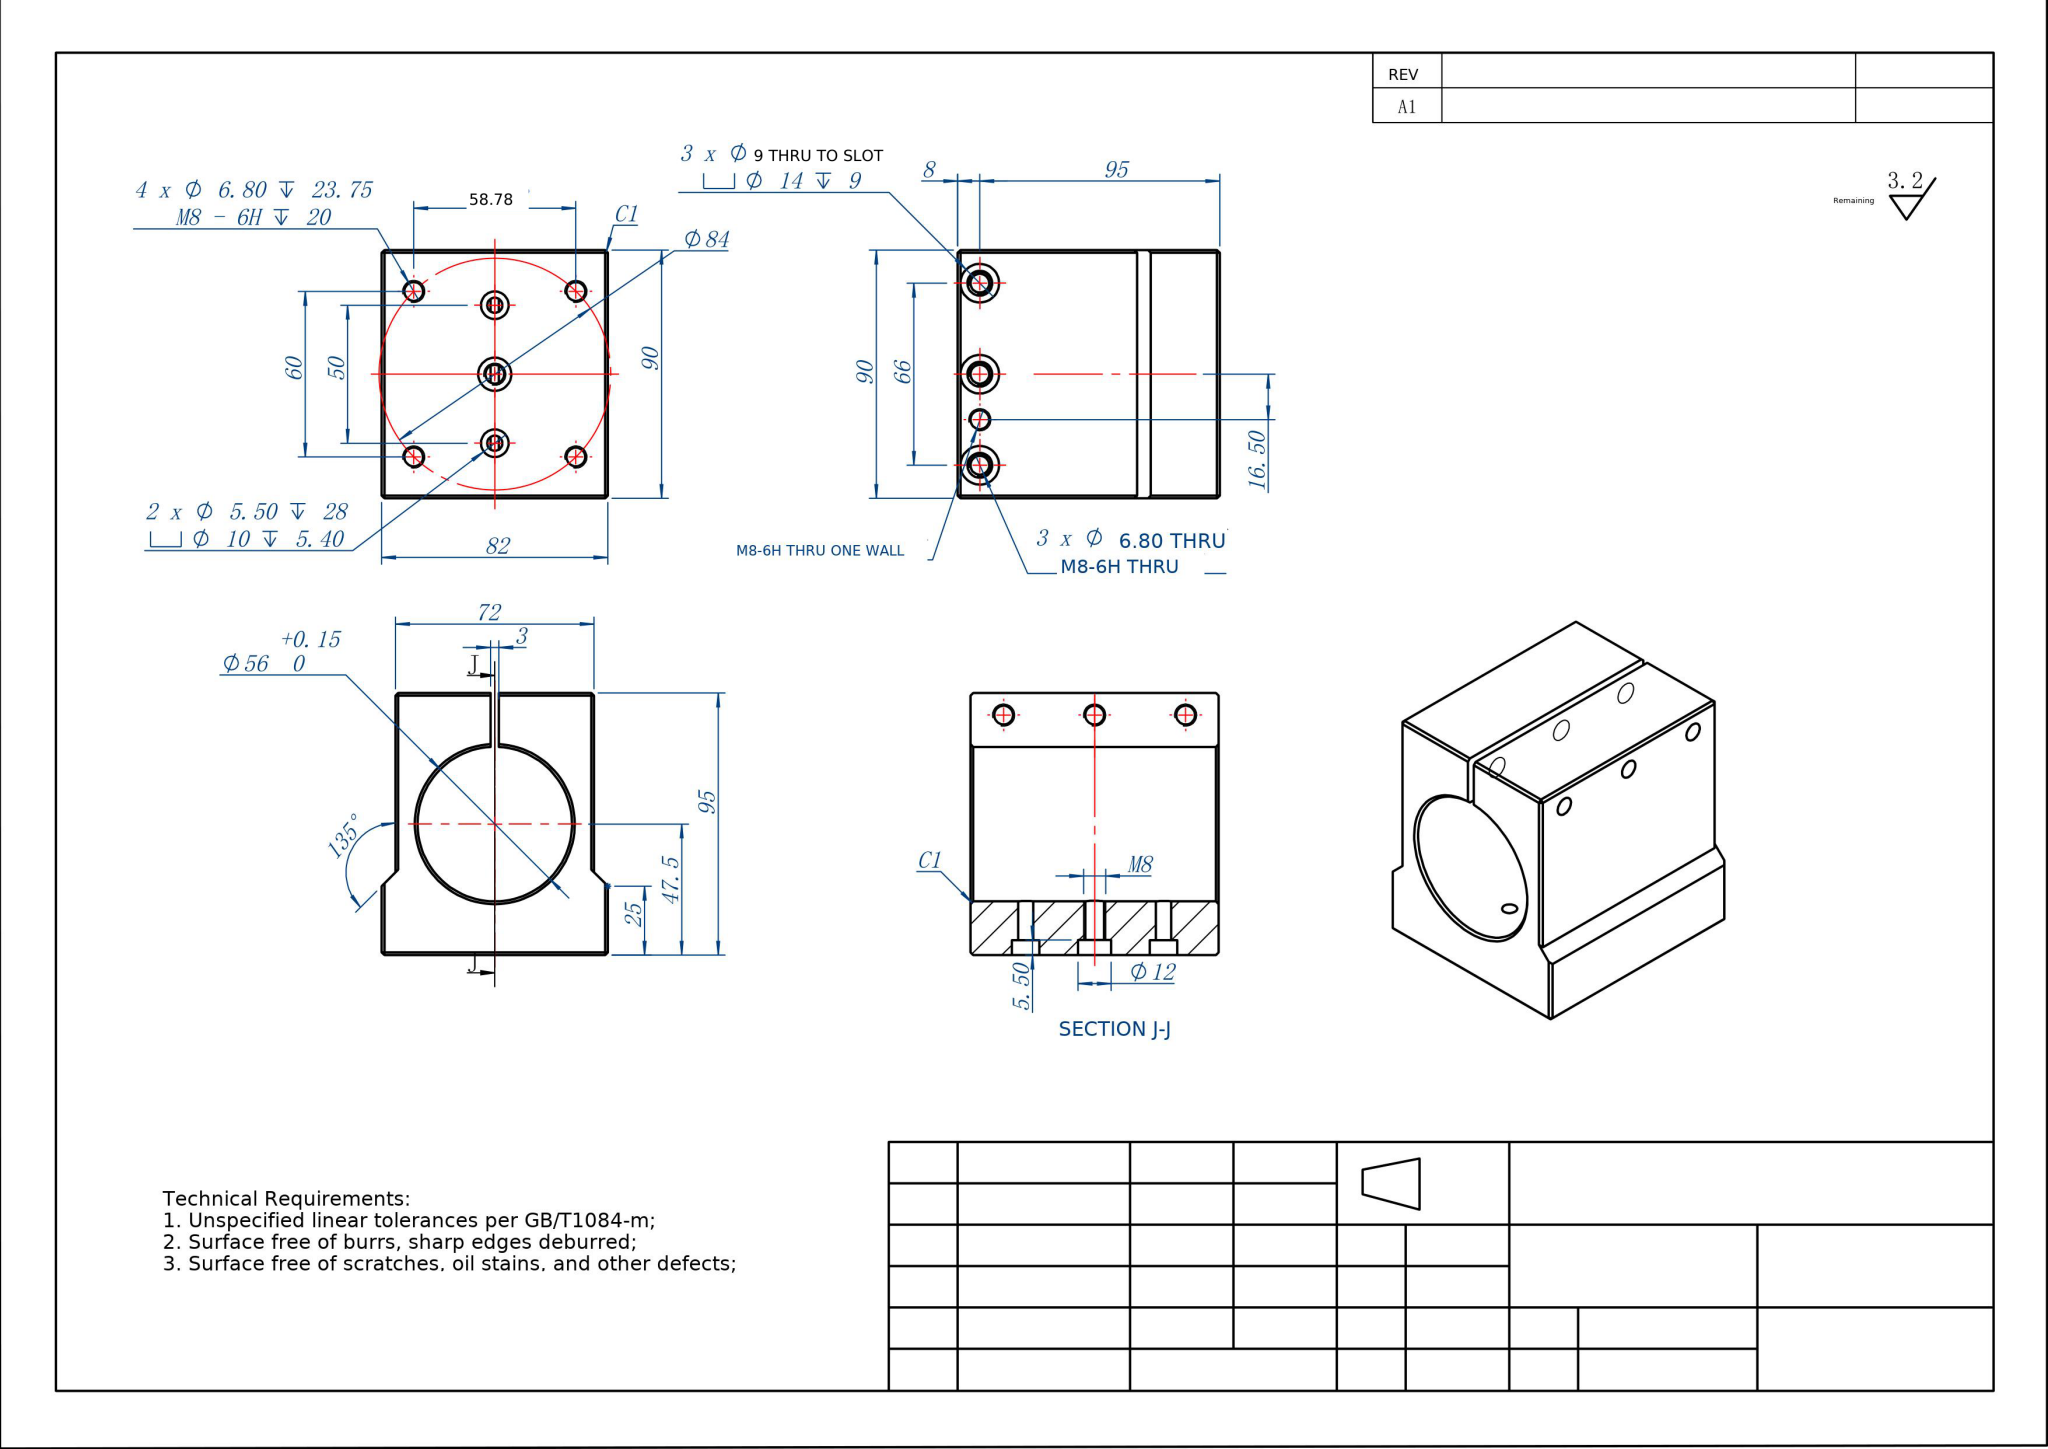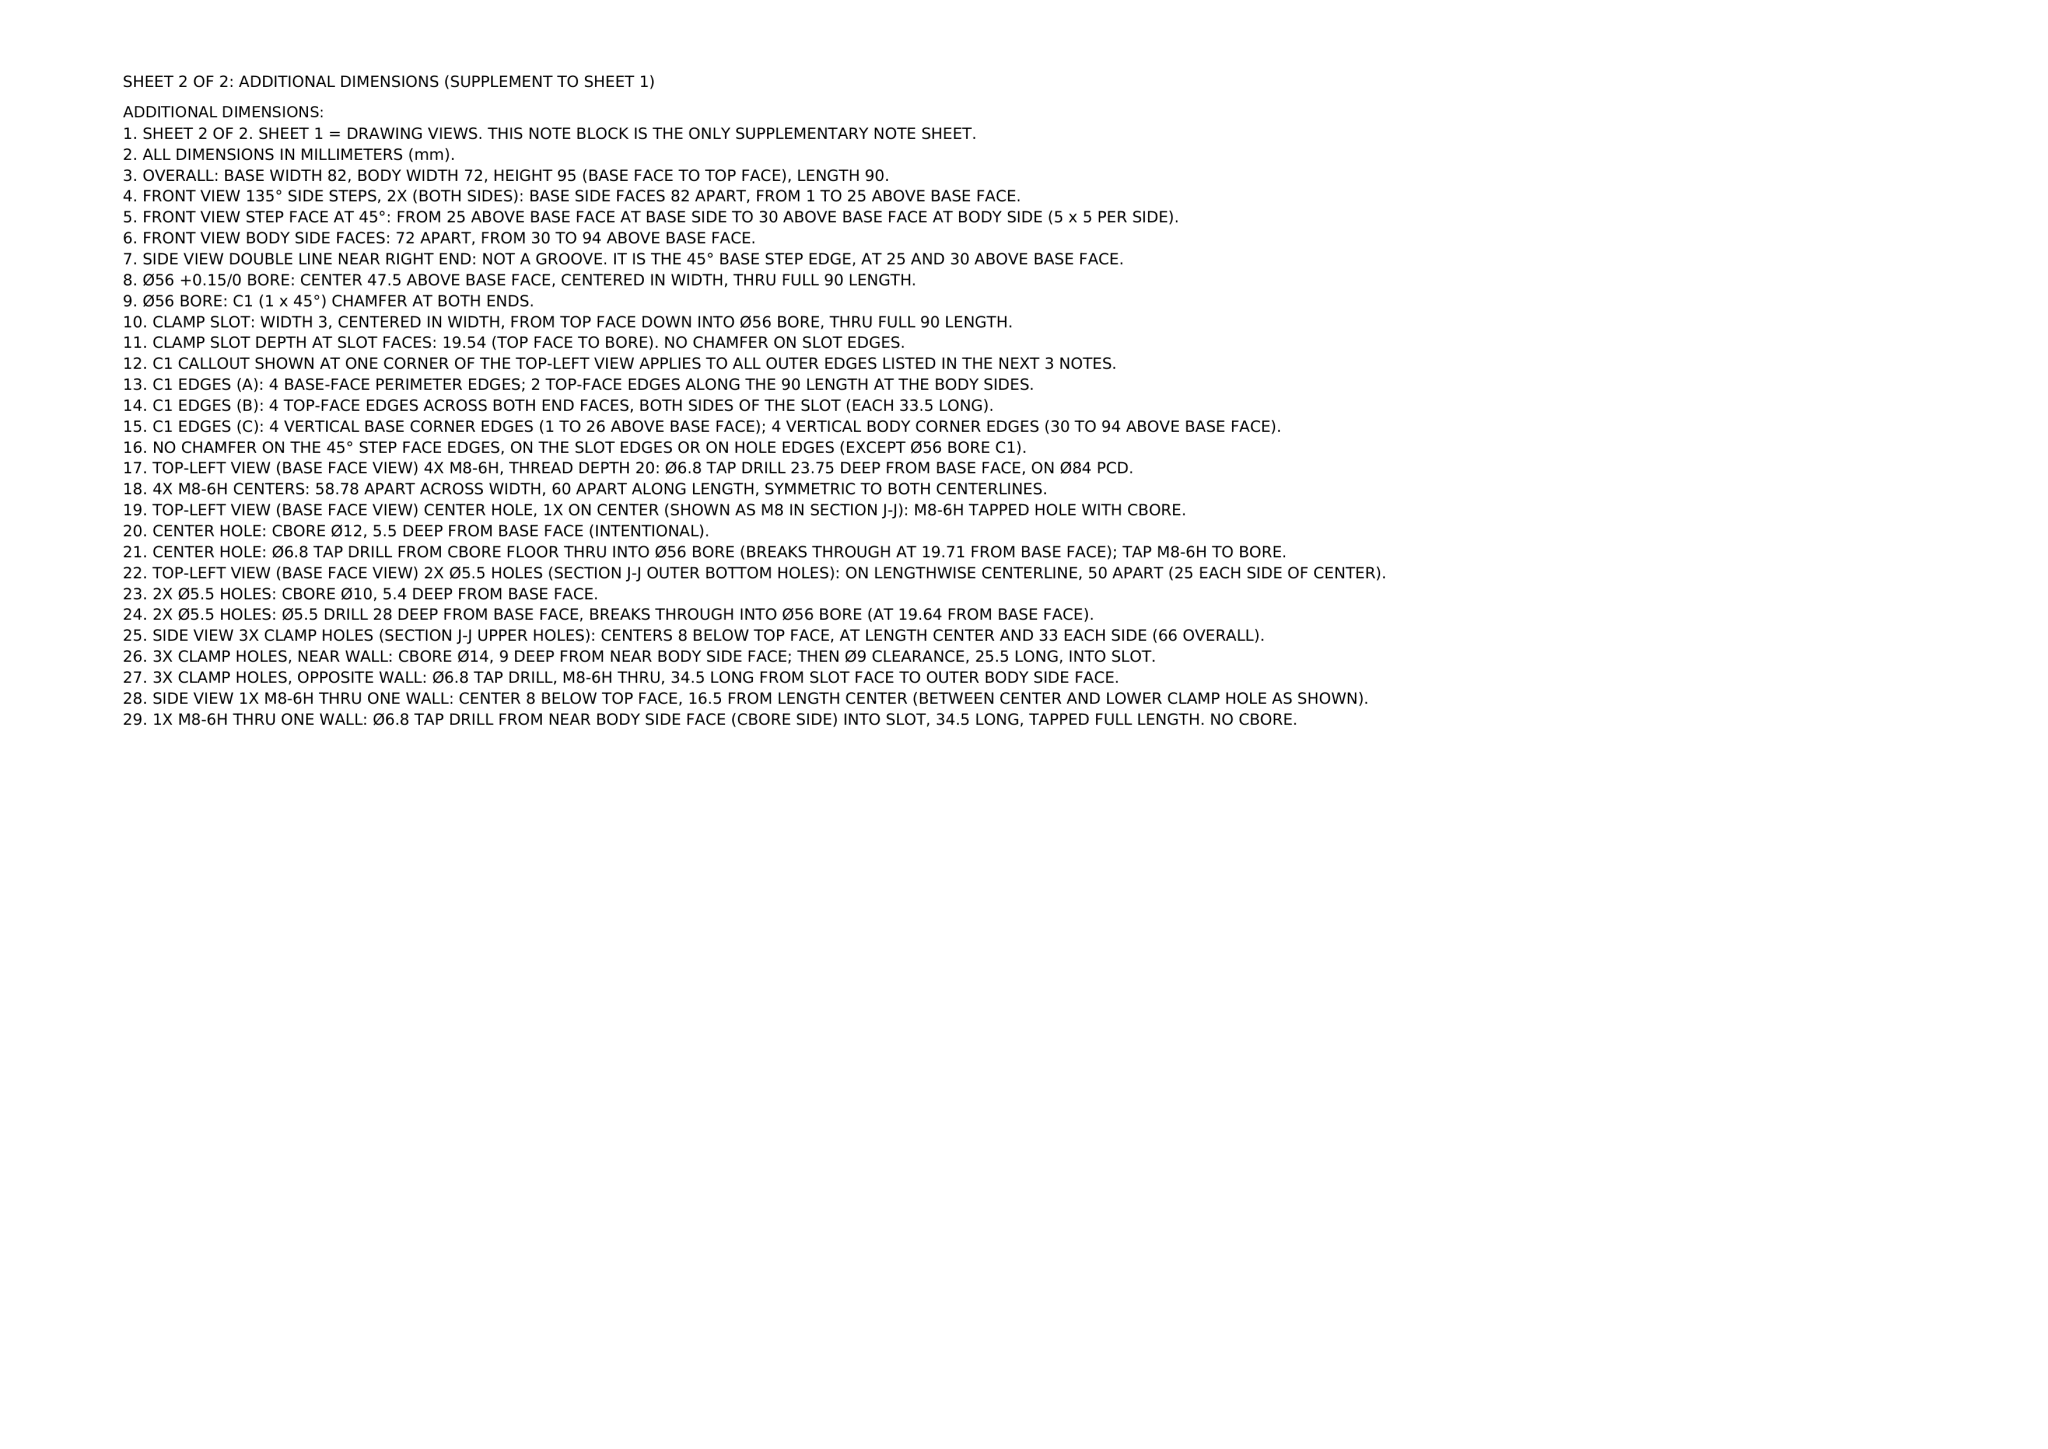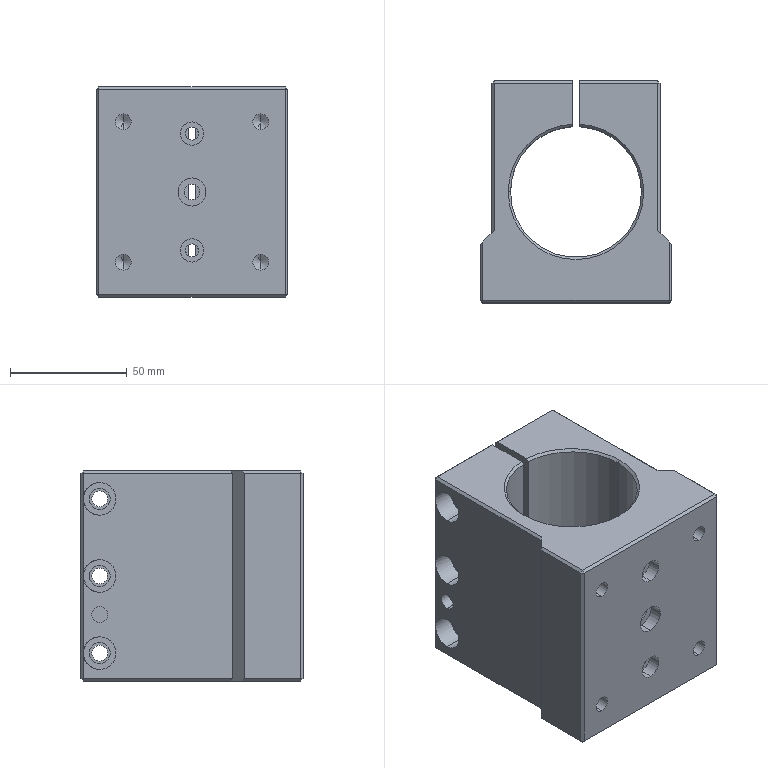Part | NX | mm | 1 solid | 102 faces | box 82 x 95 x 90 mm | volume 392494 mm3 | plane 45 | cylinder 43 | cone 14 | commonest cylinder face diameters 6.8 x18 14 x6 9 x6 10 x4 5.5 x4 56 x3 12 x2